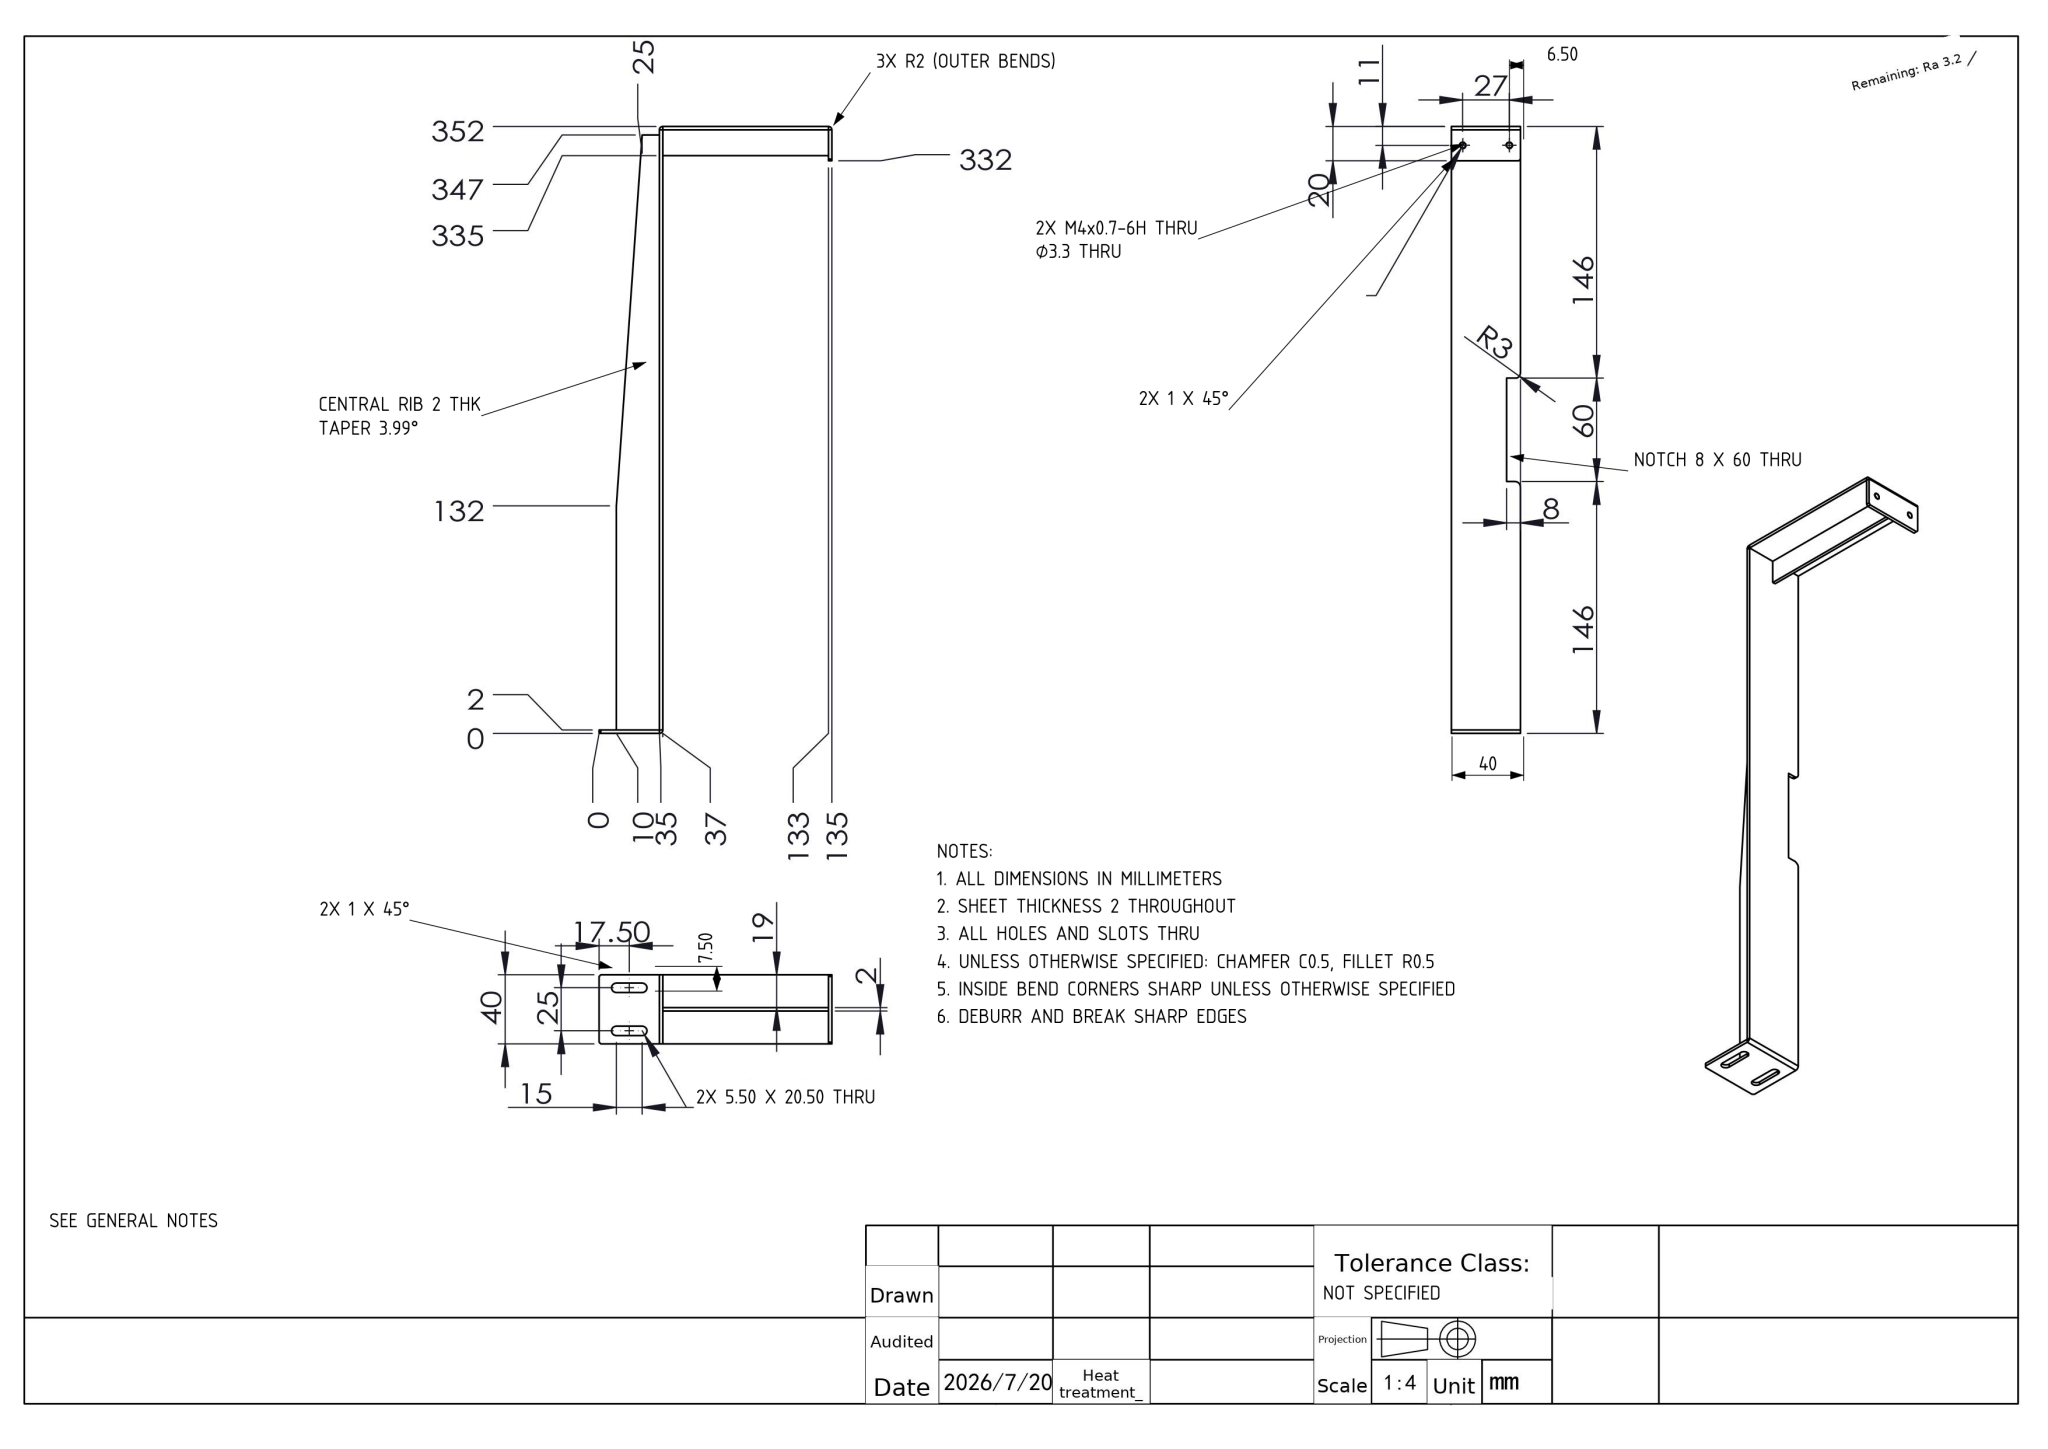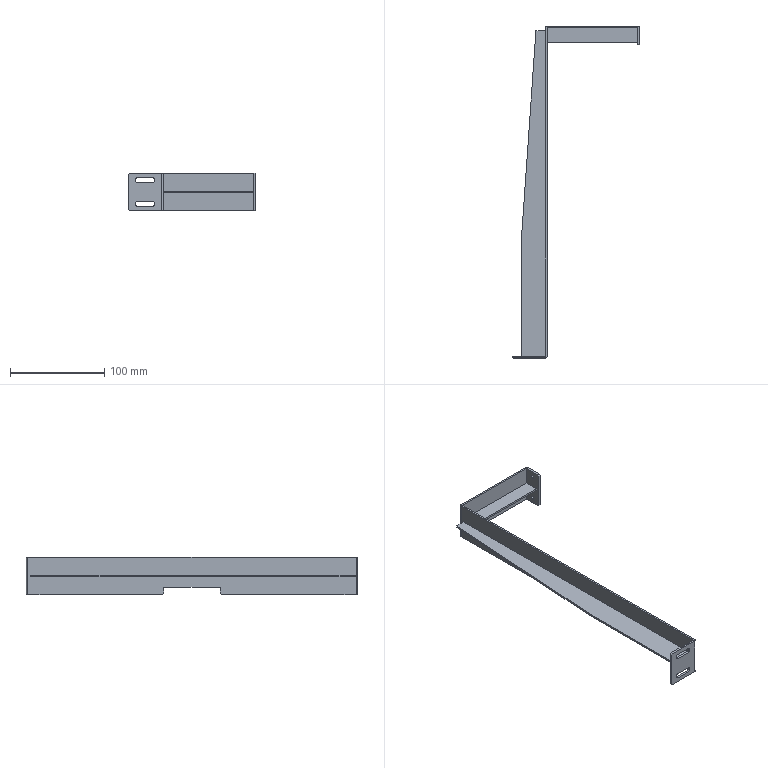Part | NX | mm | 1 solid | 58 faces | box 135 x 352 x 40 mm | volume 55611 mm3 | plane 45 | cylinder 13 | commonest cylinder face diameters 3.3 x4 5.5 x4 4 x3 6 x2